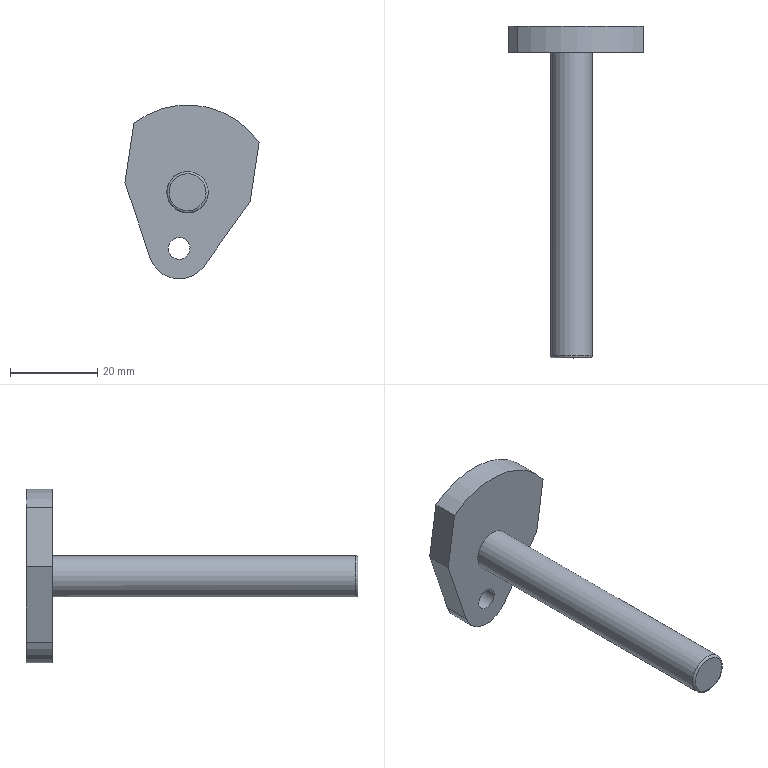Component | NX | CRANKSHAFT | 1 solid | 12 faces | volume 10205 mm3 | plane 7 | cylinder 4 | torus 1 | commonest cylinder face diameters 40 x1 14 x1 5 x1 9.5 x1